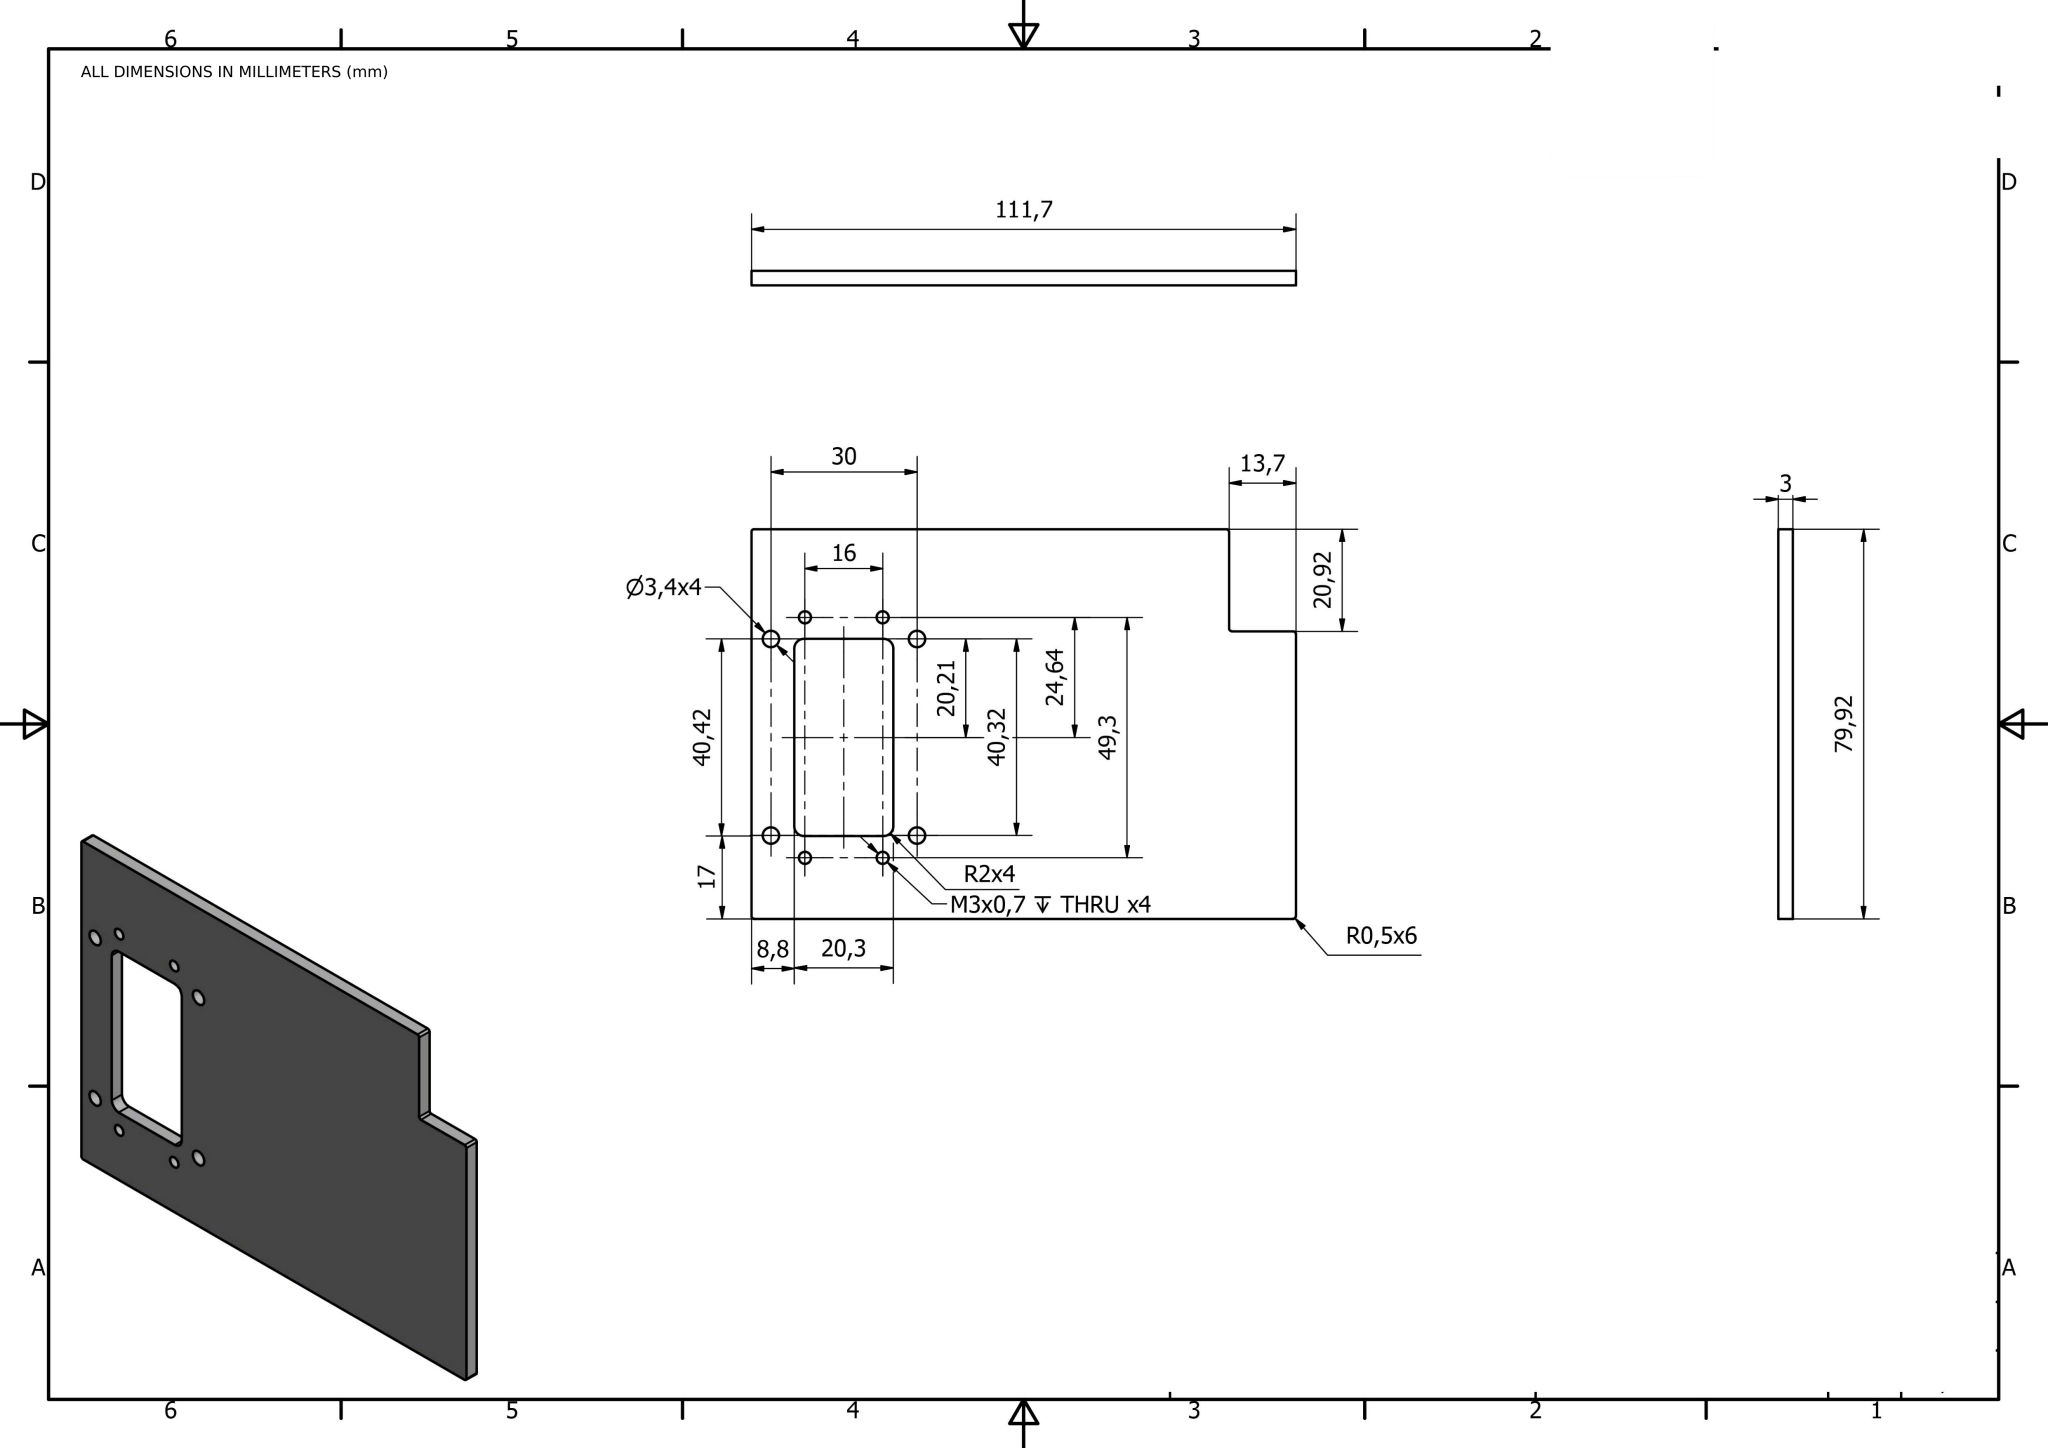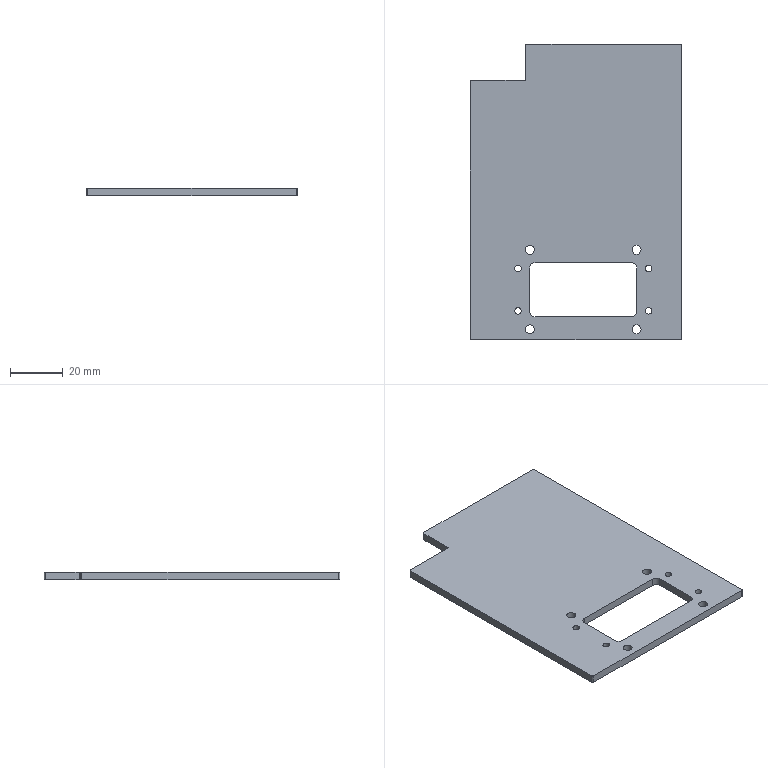Part | NX | mm | 1 solid | 30 faces | box 79.92 x 111.7 x 3 mm | volume 23302 mm3 | cylinder 18 | plane 12 | commonest cylinder face diameters 1 x6 2.5 x4 3.4 x4 4 x4